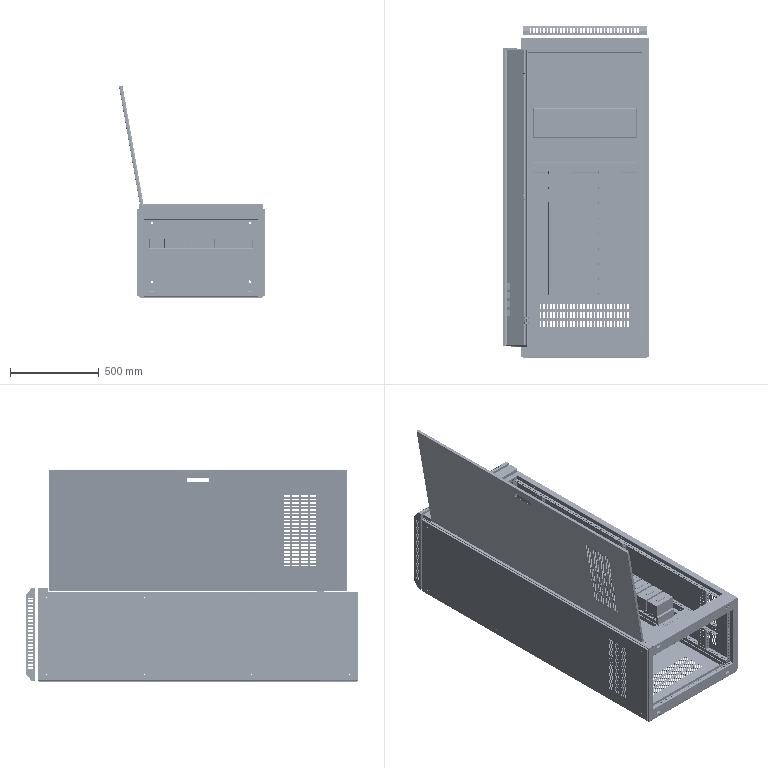Assembly | SolidWorks | mm | 45 component files | 45 solids | 9588 faces | box 820.39 x 1865.03 x 1196.61 mm | volume 18580201 mm3 | plane 5098 | cylinder 4314 | torus 128 | spline 48 | commonest cylinder face diameters 9 x3408 0.2 x288 2.6 x182 4.2 x98 4 x80 6 x52 5.1 x40 7 x40
Bill of materials:
Hinge | 1 |  | Bent sheet-metal bracket: a flat rectangular plate with a rectangular notch cut into its upper edge, which leaves two tabs. Each tab is bent over about 90 degrees and ends in a curled roll. The lower part of the plate has two obround slots side by side.
KSHE-016.004 | 2 |  | Long sheet-metal channel with an asymmetric open profile: a top web, one full-height side wall with a short inward return at its bottom, and a shorter opposite wall. There is one obround slot near each end of the full-height wall.
KSHE-016.005 | 2 |  | Long sheet-metal channel with an asymmetric profile: a top web, one full-height wall with a short return flange, and a shorter opposite wall. The top web has two small slots, and there is an obround slot near one end. At one end, a small tab carries three small round holes.
KSHE-016.006 | 6 |  | Tall rectangular hollow section, either a box or a closed channel, with regularly spaced round holes along its faces. The broad face has two columns of holes and the narrow face has one column. The end face has two obround slots.
KSHE-016.009 | 2 |  | Very long, slender C-channel (web with two flanges, rounded bends) perforated along its entire length with evenly spaced round holes in the web and in both flanges.
KSHE-016.010 | 1 |  | Hat-section sheet-metal cover: a wide flat top panel with downturned walls at both short ends, each ending in an outward flat flange with two round holes. The top panel has four small holes near its middle.
KSHE-016.011 | 2 |  | Long, shallow U-channel whose flat web extends past the side legs at both ends as flat tabs. Each tab has two round holes, and the web has four further round holes along its length.
KSHE-016.012 | 2 |  | Hat-section sheet-metal cover similar in form to a raised tray: a flat rectangular top with downturned end walls, each ending in an outward flange with two small holes. The top panel has no visible holes.
KSHE-016.014 | 2 |  | Short, shallow sheet-metal U-channel: a flat rectangular web with two short side flanges and rounded bends. There is one round hole near each end of the web.
KSHE-016.015 | 1 |  | Rectangular sheet-metal panel with flanges folded around its perimeter, forming a shallow tray. The side flanges have chamfered corner profiles. The flanges carry rows of narrow parallel slots that look like vents, and the main face has four round holes near its corners.
KSHE-016.016 | 1 |  | Long flat rectangular bar or plate. Two orthographic views show small projecting pins or stubs, including a cylindrical boss, that are not visible in the iso view.
KSHE-016.018 | 1 |  | Large thin flat rectangular sheet with three parallel rows of narrow slots grouped near one end, plus small holes spaced along the long edges.
KSHE-016.019 | 2 |  | Thin, flat, elongated rectangular plate with three parallel columns of short slots near one end, plus small holes spaced along both long edges.
KSHE-016.001 | 2 |  | Long, straight channel with an uneven C-shaped section: a web, two flanges, and a partial return lip on one flange only. A row of evenly spaced small holes runs along one face, and the ends are cut at an angle.
KSHE-016.002 | 2 |  | Long, straight channel similar to unnamed part, but with the partial return lip on the opposite flange (it may be a mirrored version). A row of small holes runs along the length, and the ends are cut at an angle.
KSHE-016.003 | 4 |  | Short channel with an uneven C-shaped section (web, two flanges, and a partial return lip on one flange). A column of small holes runs along one face, and one end appears to be cut at an angle.
Hinge1 | 1 |  | T-shaped flat plate with two parallel obround (slotted) holes in the wide part. A narrow tongue extends from it and ends in a rolled, partly open cylindrical curl.
KSHE-016.017 | 1 |  | Large, thin rectangular panel with four columns of short slots near one end, a single rectangular cutout near one long edge, and small paired holes or features along the opposite long edge.
Switch | 10 |  | Solid rectangular block with a low, raised rectangular pad on the top face and four small holes near the corners of the top face.
Mates:
1. coincident | KSHE-016.004-1 face at (-287.273, 13.814, 31.5) dir (-1, 0, 0) | KSHE-016.1.SLDPRT-1/KSHE-016.003-2 face at (-287.273, -69.186, -216.5) dir (1, 0, 0)
2. coincident | KSHE-016.004-1 face at (32.727, -28.686, 33.5) dir (0, 0, 1) | KSHE-016.1.SLDPRT-1/KSHE-016.001-1 face at (-317.273, 828.814, 33.5) dir (0, 0, 1)
3. coincident | KSHE-016.004-1 face at (32.727, -71.186, 33.5) dir (0, -1, 0) | KSHE-016.1.SLDPRT-1/KSHE-016.003-2 face at (-302.273, -71.186, -216.5) dir (0, -1, 0)
4. coincident | KSHE-016.1.SLDPRT-1/KSHE-016.002-1 face at (-317.273, 828.814, -466.5) dir (0, 0, -1) | KSHE-016.004-2 face at (32.727, -28.686, -466.5) dir (0, 0, -1)
5. coincident | KSHE-016.1.SLDPRT-1/KSHE-016.002-1 face at (-287.273, 828.814, -441.5) dir (1, 0, 0) | KSHE-016.004-2 face at (-287.273, -71.186, -399.5) dir (-1, 0, 0)
6. coincident | KSHE-016.1.SLDPRT-1/KSHE-016.003-2 face at (-302.273, -71.186, -216.5) dir (0, -1, 0) | KSHE-016.004-2 face at (32.727, -71.186, -466.5) dir (0, -1, 0)
7. coincident | KSHE-016.004-2 face at (32.727, -28.686, -466.5) dir (0, 0, -1) | KSHE-016.1.SLDPRT-2/KSHE-016.002-1 face at (382.727, 828.814, -466.5) dir (0, 0, -1)
8. coincident | KSHE-016.004-2 face at (352.727, -71.186, -464.5) dir (1, 0, 0) | KSHE-016.1.SLDPRT-2/KSHE-016.003-1 face at (352.727, -69.186, -216.5) dir (-1, 0, 0)
9. coincident | KSHE-016.004-2 face at (32.727, -71.186, -466.5) dir (0, -1, 0) | KSHE-016.1.SLDPRT-2/KSHE-016.003-1 face at (367.727, -71.186, -216.5) dir (0, -1, 0)
10. coincident | KSHE-016.1.SLDPRT-1/KSHE-016.002-1 face at (-317.273, 828.814, -466.5) dir (0, 0, -1) | KSHE-016.005-2 face at (32.727, 1686.314, -466.5) dir (0, 0, -1)
11. coincident | KSHE-016.1.SLDPRT-1/KSHE-016.003-1 face at (-302.273, 1728.814, -216.5) dir (0, 1, 0) | KSHE-016.005-2 face at (32.727, 1728.814, -466.5) dir (0, 1, 0)
12. coincident | KSHE-016.1.SLDPRT-1/KSHE-016.002-1 face at (-287.273, 828.814, -441.5) dir (1, 0, 0) | KSHE-016.005-2 face at (-287.273, 1728.814, -464.5) dir (-1, 0, 0)
13. coincident | KSHE-016.005-1 face at (32.727, 1728.814, 33.5) dir (0, 1, 0) | KSHE-016.005-2 face at (32.727, 1728.814, -466.5) dir (0, 1, 0)
14. coincident | KSHE-016.1.SLDPRT-1/KSHE-016.001-1 face at (-317.273, 828.814, 33.5) dir (0, 0, 1) | KSHE-016.005-1 face at (32.727, 1686.314, 33.5) dir (0, 0, 1)
15. coincident | KSHE-016.1.SLDPRT-1/KSHE-016.001-1 face at (-287.273, 828.814, 8.5) dir (1, 0, 0) | KSHE-016.005-1 face at (-287.273, 1643.814, 31.5) dir (-1, 0, 0)
16. distance | KSHE-016.1.SLDPRT-1/KSHE-016.001-1 face at (-317.273, 828.814, -16.5) dir (0, 0, -1) | KSHE-016.006-1 face at (-287.273, 1478.814, -18) dir (0, 0, 1)
17. coincident | KSHE-016.1.SLDPRT-2/KSHE-016.001-1 face at (352.727, 1678.814, -16.5) dir (-1, 0, 0) | KSHE-016.006-2 face at (352.727, 1478.814, -216.5) dir (-1, 0, 0)
18. coincident | KSHE-016.006-1 face at (-287.273, 1478.814, -18) dir (0, 0, 1) | KSHE-016.006-2 face at (352.727, 1478.814, -18) dir (0, 0, 1)
19. coincident | KSHE-016.006-1 face at (-287.273, 1508.814, -216.5) dir (0, 1, 0) | KSHE-016.006-2 face at (352.727, 1508.814, -216.5) dir (0, 1, 0)
20. distance | KSHE-016.006-1 face at (-287.273, 1508.814, -216.5) dir (0, 1, 0) | KSHE-016.1.SLDPRT-1/KSHE-016.003-1 face at (-302.273, 1728.814, -216.5) dir (0, 1, 0)
21. coincident | KSHE-016.1.SLDPRT-1/KSHE-016.002-1 face at (-287.273, 1678.814, -416.5) dir (1, 0, 0) | KSHE-016.006-1 face at (-287.273, 1478.814, -216.5) dir (1, 0, 0)
22. coincident | KSHE-016.006-1 face at (-287.273, 1478.814, -216.5) dir (1, 0, 0) | KSHE-016.009-2 face at (-287.273, 778.814, -226.5) dir (-1, 0, 0)
23. concentric | KSHE-016.006-1 face at (-687.273, 1488.814, -216.5) dir (1, 0, 0) r 4.5 | KSHE-016.009-2 face at (-277.273, 1488.814, -216.5) dir (-1, 0, 0) r 4.5
24. coincident | KSHE-016.1.SLDPRT-2/KSHE-016.003-2 face at (352.727, 1726.814, -216.5) dir (-1, 0, 0) | KSHE-016.014-1 face at (352.727, 1728.814, -216.5) dir (1, 0, 0)
25. coincident | KSHE-016.1.SLDPRT-2/KSHE-016.003-2 face at (367.727, 1728.814, -216.5) dir (0, 1, 0) | KSHE-016.014-1 face at (307.727, 1728.814, -216.5) dir (0, 1, 0)
26. coincident | KSHE-016.005-1 face at (32.727, 1686.314, -33.5) dir (0, 0, -1) | KSHE-016.014-1 face at (262.727, 1726.314, -33.5) dir (0, 0, 1)
27. concentric | KSHE-016.014-1 face at (307.727, 1718.814, -51.5) dir (0, 1, 0) r 8 | KSHE-016.015-1 face at (307.727, 1783.841, -51.5) dir (0, 1, 0) r 6.5
28. concentric | KSHE-016.014-2 face at (-242.273, 1718.814, -51.5) dir (0, 1, 0) r 8 | KSHE-016.015-1 face at (-242.273, 1783.841, -51.5) dir (0, 1, 0) r 6.5
29. distance | KSHE-016.014-2 face at (-242.273, 1728.814, -216.5) dir (0, 1, 0) | KSHE-016.015-1 face at (32.727, 1743.814, -206.5) dir (0, -1, 0)
30. coincident | KSHE-016.005-1 face at (32.727, 1686.314, 33.5) dir (0, 0, 1) | KSHE-016.016-1 face at (377.727, 1669.814, 33.5) dir (0, 0, -1)
31. distance | KSHE-016.005-1 face at (32.727, 1728.814, 33.5) dir (0, 1, 0) | KSHE-016.016-1 face at (32.727, 1727.814, 55.5) dir (0, 1, 0)
32. distance | KSHE-016.1.SLDPRT-2/KSHE-016.001-1 face at (382.727, 828.814, 8.5) dir (1, 0, 0) | KSHE-016.016-1 face at (377.727, 1698.814, 55.5) dir (1, 0, 0)
33. coincident | KSHE-016.012-1 face at (172.727, 629.814, -141.5) dir (0, 0, 1) | Switch-1 face at (172.727, 924.814, -141.5) dir (0, 0, -1)
34. coincident | KSHE-016.012-1 face at (107.727, 629.814, -141.5) dir (-1, 0, 0) | Switch-1 face at (107.727, 962.314, -69.5) dir (-1, 0, 0)
35. distance | KSHE-016.012-1 face at (172.727, 979.814, -141.5) dir (0, 1, 0) | Switch-1 face at (107.727, 962.314, -69.5) dir (0, 1, 0)
36. coincident | KSHE-016.006-2 face at (352.727, 1478.814, -216.5) dir (-1, 0, 0) | KSHE-016.009-3 face at (352.727, 778.814, -226.5) dir (1, 0, 0)
37. coincident | KSHE-016.009-2 face at (-287.273, 778.814, -256.5) dir (0, 0, -1) | KSHE-016.009-3 face at (352.727, 778.814, -256.5) dir (0, 0, -1)
38. concentric | KSHE-016.006-1 face at (-687.273, 1468.814, -216.5) dir (1, 0, 0) r 4.5 | KSHE-016.009-2 face at (-277.273, 1468.814, -216.5) dir (-1, 0, 0) r 4.5
39. concentric | KSHE-016.006-2 face at (752.727, 1488.814, -236.5) dir (-1, 0, 0) r 4.5 | KSHE-016.009-3 face at (342.727, 1488.814, -236.5) dir (1, 0, 0) r 4.5
40. coincident | KSHE-016.009-2 face at (-287.273, 778.814, -196.5) dir (0, 0, 1) | KSHE-016.010-2 face at (32.727, 1248.814, -196.5) dir (0, 0, -1)
41. concentric | KSHE-016.009-2 face at (-272.273, 1288.814, -256.5) dir (0, 0, 1) r 4.5 | KSHE-016.010-2 face at (-272.273, 1288.814, -186.5) dir (0, 0, -1) r 4.5
42. concentric | KSHE-016.009-2 face at (-272.273, 1208.814, -256.5) dir (0, 0, 1) r 4.5 | KSHE-016.010-2 face at (-272.273, 1208.814, -186.5) dir (0, 0, -1) r 4.5
43. coincident | KSHE-016.009-2 face at (-287.273, 778.814, -196.5) dir (0, 0, 1) | KSHE-016.011-4 face at (32.727, 998.814, -196.5) dir (0, 0, -1)
44. concentric | KSHE-016.009-2 face at (-272.273, 1008.814, -256.5) dir (0, 0, 1) r 4.5 | KSHE-016.011-4 face at (-272.273, 1008.814, -204.5) dir (0, 0, 1) r 4.5
45. concentric | KSHE-016.009-2 face at (-272.273, 988.814, -256.5) dir (0, 0, 1) r 4.5 | KSHE-016.011-4 face at (-272.273, 988.814, -204.5) dir (0, 0, 1) r 4.5
46. coincident | KSHE-016.012-1 face at (172.727, 629.814, -194.5) dir (0, 0, -1) | KSHE-016.011-4 face at (32.727, 998.814, -194.5) dir (0, 0, 1)
47. concentric | KSHE-016.012-1 face at (132.727, 998.814, -202.5) dir (0, 0, 1) r 4.5 | KSHE-016.011-4 face at (132.727, 998.814, -204.5) dir (0, 0, 1) r 4.5
48. concentric | KSHE-016.012-1 face at (212.727, 998.814, -202.5) dir (0, 0, 1) r 4.5 | KSHE-016.011-4 face at (212.727, 998.814, -204.5) dir (0, 0, 1) r 4.5
49. coincident | KSHE-016.012-3 face at (-107.273, 629.814, -141.5) dir (0, 0, 1) | Switch-9 face at (-107.273, 924.814, -141.5) dir (0, 0, -1)
50. coincident | KSHE-016.012-3 face at (-172.273, 629.814, -141.5) dir (-1, 0, 0) | Switch-9 face at (-172.273, 962.314, -69.5) dir (-1, 0, 0)
51. coincident | Switch-1 face at (107.727, 962.314, -69.5) dir (0, 1, 0) | Switch-9 face at (-172.273, 962.314, -69.5) dir (0, 1, 0)
52. coincident | KSHE-016.1.SLDPRT-1/KSHE-016.001-1 face at (-287.273, 828.814, 8.5) dir (1, 0, 0) | Hinge-2 face at (-287.273, 138.814, 32.75) dir (-1, 0, 0)
53. concentric | KSHE-016.1.SLDPRT-1/KSHE-016.001-1 face at (-297.273, 148.814, 21) dir (1, 0, 0) r 2.55 | Hinge-2 face at (-314.273, 148.814, 21) dir (1, 0, 0) r 3.5
54. concentric | KSHE-016.1.SLDPRT-1/KSHE-016.001-1 face at (-297.273, 128.814, 21) dir (1, 0, 0) r 2.55 | Hinge-2 face at (-314.273, 128.814, 21) dir (1, 0, 0) r 3.5
55. coincident | KSHE-016.1.SLDPRT-2/KSHE-016.003-1 face at (382.727, -69.186, -216.5) dir (1, 0, 0) | KSHE-016.019-1 face at (382.727, -66.186, 27.2) dir (-1, 0, 0)
56. distance | KSHE-016.1.SLDPRT-2/KSHE-016.002-1 face at (382.727, 828.814, -466.5) dir (0, 0, -1) | KSHE-016.019-1 face at (392.727, 828.814, -461.5) dir (0, 0, -1)
57. distance | KSHE-016.1.SLDPRT-2/KSHE-016.003-1 face at (367.727, -71.186, -216.5) dir (0, -1, 0) | KSHE-016.019-1 face at (392.727, -66.186, -216.5) dir (0, -1, 0)
58. coincident | KSHE-016.1.SLDPRT-1/KSHE-016.003-2 face at (-317.273, -69.186, -216.5) dir (-1, 0, 0) | KSHE-016.019-2 face at (-317.273, -66.186, -460.2) dir (1, 0, 0)
59. distance | KSHE-016.1.SLDPRT-1/KSHE-016.001-1 face at (-317.273, 828.814, 33.5) dir (0, 0, 1) | KSHE-016.019-2 face at (-327.273, 828.814, 28.5) dir (0, 0, 1)
60. distance | KSHE-016.019-2 face at (-327.273, -66.186, -216.5) dir (0, -1, 0) | KSHE-016.1.SLDPRT-1/KSHE-016.003-2 face at (-302.273, -71.186, -216.5) dir (0, -1, 0)
61. coincident | KSHE-016.1.SLDPRT-1/KSHE-016.002-1 face at (-317.273, 828.814, -466.5) dir (0, 0, -1) | KSHE-016.018-1 face at (376.427, -66.186, -466.5) dir (0, 0, 1)
62. distance | KSHE-016.018-1 face at (-312.273, 828.814, -476.5) dir (-1, 0, 0) | KSHE-016.1.SLDPRT-1/KSHE-016.002-1 face at (-317.273, 828.814, -441.5) dir (-1, 0, 0)
63. distance | KSHE-016.004-2 face at (32.727, -71.186, -466.5) dir (0, -1, 0) | KSHE-016.018-1 face at (32.727, -66.186, -476.5) dir (0, -1, 0)
64. concentric | Hinge-2 face at (-302.773, 158.814, 48.5) dir (0, 1, 0) r 5.5 | KSHE-016.4-1/Hinge1-1 face at (-302.773, 148.814, 48.5) dir (0, 1, 0) r 5.5
65. distance | Hinge-2 face at (-314.273, 128.814, 61.053) dir (0, 1, 0) | KSHE-016.4-1/Hinge1-1 face at (-302.773, 129.814, 48.5) dir (0, -1, 0)
66. angle | KSHE-016.4-1/KSHE-016.017-1 face at (-368.013, 829.314, 378.18) dir (-0.9848, 0, -0.1736) | KSHE-016.016-1 face at (32.727, 1698.814, 55.5) dir (0, 0, 1)
67. coincident | KSHE-016.001-1 face at (-196.624, 62.511, 15) dir (0, 0, 1) | KSHE-016.003-1 face at (701.376, 287.511, 15) dir (0, 0, 1)
68. coincident | KSHE-016.001-1 face at (703.376, 37.511, -15) dir (1, 0, 0) | KSHE-016.003-1 face at (703.376, 287.511, 0) dir (1, 0, 0)
69. coincident | KSHE-016.001-1 face at (-196.624, 39.511, 15) dir (0, 1, 0) | KSHE-016.003-1 face at (703.376, 39.511, 15) dir (0, -1, 0)
70. coincident | KSHE-016.003-1 face at (701.376, 287.511, 15) dir (0, 0, 1) | KSHE-016.002-1 face at (-196.624, 512.511, 15) dir (0, 0, 1)
71. coincident | KSHE-016.003-1 face at (703.376, 535.511, 15) dir (0, 1, 0) | KSHE-016.002-1 face at (-196.624, 535.511, 15) dir (0, -1, 0)
72. coincident | KSHE-016.003-1 face at (703.376, 287.511, 0) dir (1, 0, 0) | KSHE-016.002-1 face at (703.376, 537.511, 13) dir (1, 0, 0)
73. coincident | KSHE-016.002-1 face at (-196.624, 512.511, 15) dir (0, 0, 1) | KSHE-016.003-2 face at (-1094.624, 287.511, 15) dir (0, 0, 1)
74. coincident | KSHE-016.002-1 face at (-1096.624, 537.511, -15) dir (-1, 0, 0) | KSHE-016.003-2 face at (-1096.624, 287.511, 0) dir (-1, 0, 0)
75. coincident | KSHE-016.001-1 face at (-196.624, 39.511, 15) dir (0, 1, 0) | KSHE-016.003-2 face at (-1096.624, 39.511, 15) dir (0, -1, 0)
76. coincident | KSHE-016.017-1 face at (177.478, -24.154, 8.536) dir (0, 0, -1) | Hinge1-1 face at (867.478, -340.154, 8.536) dir (0, 0, 1)
77. concentric | KSHE-016.017-1 face at (877.478, -325.154, -3.464) dir (0, 0, 1) r 3 | Hinge1-1 face at (877.478, -325.154, -1.464) dir (0, 0, 1) r 3.5
78. concentric | KSHE-016.017-1 face at (857.478, -325.154, -3.464) dir (0, 0, 1) r 3 | Hinge1-1 face at (857.478, -325.154, -1.464) dir (0, 0, 1) r 3.5